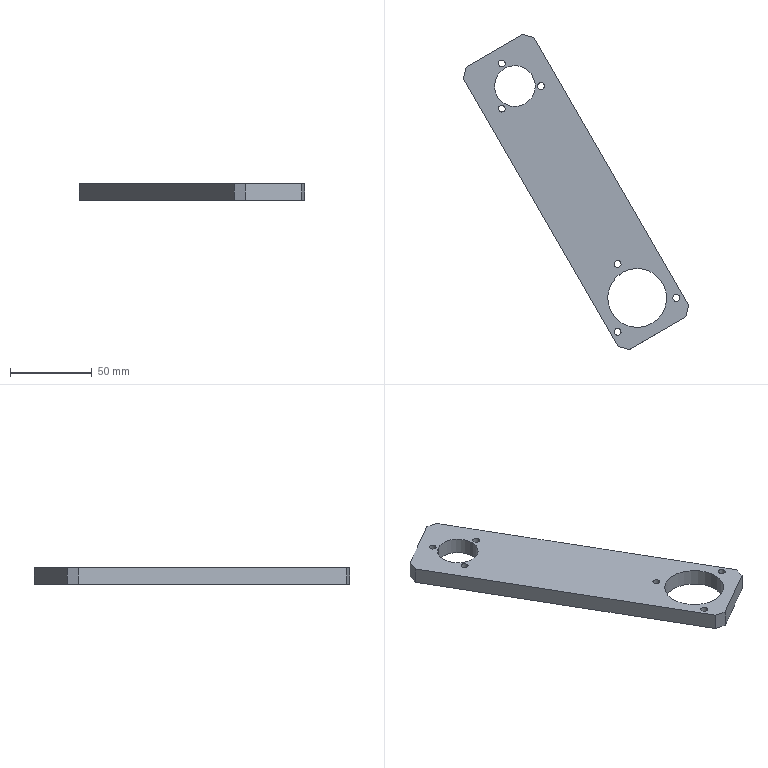Component | SolidWorks | JYTBJ-HeaderPlateSupportFrameA-1 | 1 solid | 26 faces | box 138.3 x 193.21 x 10 mm | volume 83525 mm3 | cylinder 16 | plane 10 | commonest cylinder face diameters 4.2 x12 36.1 x2 25 x2
build123d program:
from build123d import *

# Parameters (mm, degrees)
SKETCH1_W           = 200
SKETCH1_H           = 50
SKETCH1_R           = 12.5
SKETCH1_R_2         = 18.05
BOSS_EXTRUDE1_DEPTH = 10
M5_TAPPED_HOLE1_D   = 4.2
CIRPATTERN1_COUNT   = 3
M5_TAPPED_HOLE2_D   = 4.2
CIRPATTERN2_COUNT   = 3
CHAMFER1_SIZE       = 5


with BuildPart() as part:
    # Sketch1 → Boss-Extrude1 (new body)
    with BuildSketch(Plane.XY):
        with Locations((75, 0)):
            Rectangle(SKETCH1_W, SKETCH1_H)
        Circle(SKETCH1_R, mode=Mode.SUBTRACT)
        with Locations((150, 0)):
            Circle(SKETCH1_R_2, mode=Mode.SUBTRACT)
    extrude(amount=BOSS_EXTRUDE1_DEPTH)

    # M5 Tapped Hole1 (through all)
    with Locations(Plane.XY.offset(10)):
        with Locations((126, 0)):
            m5_tapped_hole1 = Hole(M5_TAPPED_HOLE1_D / 2)

    # CirPattern1: M5 Tapped Hole1 ×3 about axis
    cirpattern1_axis = Axis((150, 0, 0), (0, 0, 1))
    for i in range(1, CIRPATTERN1_COUNT):
        add(m5_tapped_hole1.rotate(cirpattern1_axis, i * 360 / CIRPATTERN1_COUNT), mode=Mode.SUBTRACT)

    # M5 Tapped Hole2 (through all)
    with Locations(Plane.XY.offset(10)):
        with Locations((-16, 0)):
            m5_tapped_hole2 = Hole(M5_TAPPED_HOLE2_D / 2)

    # CirPattern2: M5 Tapped Hole2 ×3 about axis
    cirpattern2_axis = Axis((0, 0, 0), (0, 0, 1))
    for i in range(1, CIRPATTERN2_COUNT):
        add(m5_tapped_hole2.rotate(cirpattern2_axis, i * 360 / CIRPATTERN2_COUNT), mode=Mode.SUBTRACT)

    # Chamfer1
    chamfer1_edges = [part.edges().sort_by_distance(p)[0] for p in [
        (175, -25, 5),
        (-25, -25, 5),
        (-25, 25, 5),
        (175, 25, 5),
    ]]
    chamfer(chamfer1_edges, length=CHAMFER1_SIZE)


solid = part.part

# Placed as in the assembly
solid = solid.moved(Location((-71.627, 226.781, -28), (0, 0, -60)))
STEP:
#1=CARTESIAN_POINT('',(-3.176,8.454,-1.102));
#2=VERTEX_POINT('',#1);
#3=CARTESIAN_POINT('',(-3.094,8.311,-1.102));
#4=VERTEX_POINT('',#3);
#5=CARTESIAN_POINT('',(-3.135,8.383,-1.102));
#6=DIRECTION('',(0.,0.,1.));
#7=DIRECTION('',(0.5,-0.866,0.));
#8=AXIS2_PLACEMENT_3D('',#5,#6,#7);
#9=CIRCLE('',#8,0.08268);
#10=EDGE_CURVE('',#2,#4,#9,.T.);
#11=ORIENTED_EDGE('',*,*,#10,.F.);
#12=CARTESIAN_POINT('',(-3.176,8.454,-0.7087));
#13=VERTEX_POINT('',#12);
#14=CARTESIAN_POINT('',(-3.176,8.454,-0.7087));
#15=DIRECTION('',(0.,0.,1.));
#16=VECTOR('',#15,39.37);
#17=LINE('',#14,#16);
#18=EDGE_CURVE('',#2,#13,#17,.T.);
#19=ORIENTED_EDGE('',*,*,#18,.T.);
#20=CARTESIAN_POINT('',(-3.094,8.311,-0.7087));
#21=VERTEX_POINT('',#20);
#22=CARTESIAN_POINT('',(-3.135,8.383,-0.7087));
#23=DIRECTION('',(0.,0.,1.));
#24=DIRECTION('',(0.5,-0.866,0.));
#25=AXIS2_PLACEMENT_3D('',#22,#23,#24);
#26=CIRCLE('',#25,0.08268);
#27=EDGE_CURVE('',#13,#21,#26,.T.);
#28=ORIENTED_EDGE('',*,*,#27,.T.);
#29=CARTESIAN_POINT('',(-3.094,8.311,-0.7087));
#30=DIRECTION('',(0.,0.,1.));
#31=VECTOR('',#30,39.37);
#32=LINE('',#29,#31);
#33=EDGE_CURVE('',#4,#21,#32,.T.);
#34=ORIENTED_EDGE('',*,*,#33,.F.);
#35=EDGE_LOOP('',(#11,#19,#28,#34));
#36=FACE_OUTER_BOUND('',#35,.T.);
#37=CARTESIAN_POINT('',(-3.135,8.383,-0.7087));
#38=DIRECTION('',(0.,0.,1.));
#39=DIRECTION('',(0.5,-0.866,0.));
#40=AXIS2_PLACEMENT_3D('',#37,#38,#39);
#41=CYLINDRICAL_SURFACE('',#40,0.08268);
#42=ADVANCED_FACE('',(#36),#41,.F.);
#43=CARTESIAN_POINT('',(-2.231,9.,-1.102));
#44=VERTEX_POINT('',#43);
#45=CARTESIAN_POINT('',(-2.149,8.857,-1.102));
#46=VERTEX_POINT('',#45);
#47=CARTESIAN_POINT('',(-2.19,8.928,-1.102));
#48=DIRECTION('',(0.,0.,1.));
#49=DIRECTION('',(0.5,-0.866,0.));
#50=AXIS2_PLACEMENT_3D('',#47,#48,#49);
#51=CIRCLE('',#50,0.08268);
#52=EDGE_CURVE('',#44,#46,#51,.T.);
#53=ORIENTED_EDGE('',*,*,#52,.F.);
#54=CARTESIAN_POINT('',(-2.231,9.,-0.7087));
#55=VERTEX_POINT('',#54);
#56=CARTESIAN_POINT('',(-2.231,9.,-0.7087));
#57=DIRECTION('',(0.,0.,1.));
#58=VECTOR('',#57,39.37);
#59=LINE('',#56,#58);
#60=EDGE_CURVE('',#44,#55,#59,.T.);
#61=ORIENTED_EDGE('',*,*,#60,.T.);
#62=CARTESIAN_POINT('',(-2.149,8.857,-0.7087));
#63=VERTEX_POINT('',#62);
#64=CARTESIAN_POINT('',(-2.19,8.928,-0.7087));
#65=DIRECTION('',(0.,0.,1.));
#66=DIRECTION('',(0.5,-0.866,0.));
#67=AXIS2_PLACEMENT_3D('',#64,#65,#66);
#68=CIRCLE('',#67,0.08268);
#69=EDGE_CURVE('',#55,#63,#68,.T.);
#70=ORIENTED_EDGE('',*,*,#69,.T.);
#71=CARTESIAN_POINT('',(-2.149,8.857,-0.7087));
#72=DIRECTION('',(0.,0.,1.));
#73=VECTOR('',#72,39.37);
#74=LINE('',#71,#73);
#75=EDGE_CURVE('',#46,#63,#74,.T.);
#76=ORIENTED_EDGE('',*,*,#75,.F.);
#77=EDGE_LOOP('',(#53,#61,#70,#76));
#78=FACE_OUTER_BOUND('',#77,.T.);
#79=CARTESIAN_POINT('',(-2.19,8.928,-0.7087));
#80=DIRECTION('',(0.,0.,1.));
#81=DIRECTION('',(0.5,-0.866,0.));
#82=AXIS2_PLACEMENT_3D('',#79,#80,#81);
#83=CYLINDRICAL_SURFACE('',#82,0.08268);
#84=ADVANCED_FACE('',(#78),#83,.F.);
#85=CARTESIAN_POINT('',(-3.176,9.546,-1.102));
#86=VERTEX_POINT('',#85);
#87=CARTESIAN_POINT('',(-3.094,9.402,-1.102));
#88=VERTEX_POINT('',#87);
#89=CARTESIAN_POINT('',(-3.135,9.474,-1.102));
#90=DIRECTION('',(0.,0.,1.));
#91=DIRECTION('',(0.5,-0.866,0.));
#92=AXIS2_PLACEMENT_3D('',#89,#90,#91);
#93=CIRCLE('',#92,0.08268);
#94=EDGE_CURVE('',#86,#88,#93,.T.);
#95=ORIENTED_EDGE('',*,*,#94,.F.);
#96=CARTESIAN_POINT('',(-3.176,9.546,-0.7087));
#97=VERTEX_POINT('',#96);
#98=CARTESIAN_POINT('',(-3.176,9.546,-0.7087));
#99=DIRECTION('',(0.,0.,1.));
#100=VECTOR('',#99,39.37);
#101=LINE('',#98,#100);
#102=EDGE_CURVE('',#86,#97,#101,.T.);
#103=ORIENTED_EDGE('',*,*,#102,.T.);
#104=CARTESIAN_POINT('',(-3.094,9.402,-0.7087));
#105=VERTEX_POINT('',#104);
#106=CARTESIAN_POINT('',(-3.135,9.474,-0.7087));
#107=DIRECTION('',(0.,0.,1.));
#108=DIRECTION('',(0.5,-0.866,0.));
#109=AXIS2_PLACEMENT_3D('',#106,#107,#108);
#110=CIRCLE('',#109,0.08268);
#111=EDGE_CURVE('',#97,#105,#110,.T.);
#112=ORIENTED_EDGE('',*,*,#111,.T.);
#113=CARTESIAN_POINT('',(-3.094,9.402,-0.7087));
#114=DIRECTION('',(0.,0.,1.));
#115=VECTOR('',#114,39.37);
#116=LINE('',#113,#115);
#117=EDGE_CURVE('',#88,#105,#116,.T.);
#118=ORIENTED_EDGE('',*,*,#117,.F.);
#119=EDGE_LOOP('',(#95,#103,#112,#118));
#120=FACE_OUTER_BOUND('',#119,.T.);
#121=CARTESIAN_POINT('',(-3.135,9.474,-0.7087));
#122=DIRECTION('',(0.,0.,1.));
#123=DIRECTION('',(0.5,-0.866,0.));
#124=AXIS2_PLACEMENT_3D('',#121,#122,#123);
#125=CYLINDRICAL_SURFACE('',#124,0.08268);
#126=ADVANCED_FACE('',(#120),#125,.F.);
#127=CARTESIAN_POINT('',(1.036,3.886,-1.102));
#128=VERTEX_POINT('',#127);
#129=CARTESIAN_POINT('',(1.119,3.742,-1.102));
#130=VERTEX_POINT('',#129);
#131=CARTESIAN_POINT('',(1.078,3.814,-1.102));
#132=DIRECTION('',(0.,0.,1.));
#133=DIRECTION('',(0.5,-0.866,0.));
#134=AXIS2_PLACEMENT_3D('',#131,#132,#133);
#135=CIRCLE('',#134,0.08268);
#136=EDGE_CURVE('',#128,#130,#135,.T.);
#137=ORIENTED_EDGE('',*,*,#136,.F.);
#138=CARTESIAN_POINT('',(1.036,3.886,-0.7087));
#139=VERTEX_POINT('',#138);
#140=CARTESIAN_POINT('',(1.036,3.886,-0.7087));
#141=DIRECTION('',(0.,0.,1.));
#142=VECTOR('',#141,39.37);
#143=LINE('',#140,#142);
#144=EDGE_CURVE('',#128,#139,#143,.T.);
#145=ORIENTED_EDGE('',*,*,#144,.T.);
#146=CARTESIAN_POINT('',(1.119,3.742,-0.7087));
#147=VERTEX_POINT('',#146);
#148=CARTESIAN_POINT('',(1.078,3.814,-0.7087));
#149=DIRECTION('',(0.,0.,1.));
#150=DIRECTION('',(0.5,-0.866,0.));
#151=AXIS2_PLACEMENT_3D('',#148,#149,#150);
#152=CIRCLE('',#151,0.08268);
#153=EDGE_CURVE('',#139,#147,#152,.T.);
#154=ORIENTED_EDGE('',*,*,#153,.T.);
#155=CARTESIAN_POINT('',(1.119,3.742,-0.7087));
#156=DIRECTION('',(0.,0.,1.));
#157=VECTOR('',#156,39.37);
#158=LINE('',#155,#157);
#159=EDGE_CURVE('',#130,#147,#158,.T.);
#160=ORIENTED_EDGE('',*,*,#159,.F.);
#161=EDGE_LOOP('',(#137,#145,#154,#160));
#162=FACE_OUTER_BOUND('',#161,.T.);
#163=CARTESIAN_POINT('',(1.078,3.814,-0.7087));
#164=DIRECTION('',(0.,0.,1.));
#165=DIRECTION('',(0.5,-0.866,0.));
#166=AXIS2_PLACEMENT_3D('',#163,#164,#165);
#167=CYLINDRICAL_SURFACE('',#166,0.08268);
#168=ADVANCED_FACE('',(#162),#167,.F.);
#169=CARTESIAN_POINT('',(-0.381,3.067,-1.102));
#170=VERTEX_POINT('',#169);
#171=CARTESIAN_POINT('',(-0.2983,2.924,-1.102));
#172=VERTEX_POINT('',#171);
#173=CARTESIAN_POINT('',(-0.3396,2.996,-1.102));
#174=DIRECTION('',(0.,0.,1.));
#175=DIRECTION('',(0.5,-0.866,0.));
#176=AXIS2_PLACEMENT_3D('',#173,#174,#175);
#177=CIRCLE('',#176,0.08268);
#178=EDGE_CURVE('',#170,#172,#177,.T.);
#179=ORIENTED_EDGE('',*,*,#178,.F.);
#180=CARTESIAN_POINT('',(-0.381,3.067,-0.7087));
#181=VERTEX_POINT('',#180);
#182=CARTESIAN_POINT('',(-0.381,3.067,-0.7087));
#183=DIRECTION('',(0.,0.,1.));
#184=VECTOR('',#183,39.37);
#185=LINE('',#182,#184);
#186=EDGE_CURVE('',#170,#181,#185,.T.);
#187=ORIENTED_EDGE('',*,*,#186,.T.);
#188=CARTESIAN_POINT('',(-0.2983,2.924,-0.7087));
#189=VERTEX_POINT('',#188);
#190=CARTESIAN_POINT('',(-0.3396,2.996,-0.7087));
#191=DIRECTION('',(0.,0.,1.));
#192=DIRECTION('',(0.5,-0.866,0.));
#193=AXIS2_PLACEMENT_3D('',#190,#191,#192);
#194=CIRCLE('',#193,0.08268);
#195=EDGE_CURVE('',#181,#189,#194,.T.);
#196=ORIENTED_EDGE('',*,*,#195,.T.);
#197=CARTESIAN_POINT('',(-0.2983,2.924,-0.7087));
#198=DIRECTION('',(0.,0.,1.));
#199=VECTOR('',#198,39.37);
#200=LINE('',#197,#199);
#201=EDGE_CURVE('',#172,#189,#200,.T.);
#202=ORIENTED_EDGE('',*,*,#201,.F.);
#203=EDGE_LOOP('',(#179,#187,#196,#202));
#204=FACE_OUTER_BOUND('',#203,.T.);
#205=CARTESIAN_POINT('',(-0.3396,2.996,-0.7087));
#206=DIRECTION('',(0.,0.,1.));
#207=DIRECTION('',(0.5,-0.866,0.));
#208=AXIS2_PLACEMENT_3D('',#205,#206,#207);
#209=CYLINDRICAL_SURFACE('',#208,0.08268);
#210=ADVANCED_FACE('',(#204),#209,.F.);
#211=CARTESIAN_POINT('',(-0.381,4.704,-1.102));
#212=VERTEX_POINT('',#211);
#213=CARTESIAN_POINT('',(-0.2983,4.561,-1.102));
#214=VERTEX_POINT('',#213);
#215=CARTESIAN_POINT('',(-0.3396,4.632,-1.102));
#216=DIRECTION('',(0.,0.,1.));
#217=DIRECTION('',(0.5,-0.866,0.));
#218=AXIS2_PLACEMENT_3D('',#215,#216,#217);
#219=CIRCLE('',#218,0.08268);
#220=EDGE_CURVE('',#212,#214,#219,.T.);
#221=ORIENTED_EDGE('',*,*,#220,.F.);
#222=CARTESIAN_POINT('',(-0.381,4.704,-0.7087));
#223=VERTEX_POINT('',#222);
#224=CARTESIAN_POINT('',(-0.381,4.704,-0.7087));
#225=DIRECTION('',(0.,0.,1.));
#226=VECTOR('',#225,39.37);
#227=LINE('',#224,#226);
#228=EDGE_CURVE('',#212,#223,#227,.T.);
#229=ORIENTED_EDGE('',*,*,#228,.T.);
#230=CARTESIAN_POINT('',(-0.2983,4.561,-0.7087));
#231=VERTEX_POINT('',#230);
#232=CARTESIAN_POINT('',(-0.3396,4.632,-0.7087));
#233=DIRECTION('',(0.,0.,1.));
#234=DIRECTION('',(0.5,-0.866,0.));
#235=AXIS2_PLACEMENT_3D('',#232,#233,#234);
#236=CIRCLE('',#235,0.08268);
#237=EDGE_CURVE('',#223,#231,#236,.T.);
#238=ORIENTED_EDGE('',*,*,#237,.T.);
#239=CARTESIAN_POINT('',(-0.2983,4.561,-0.7087));
#240=DIRECTION('',(0.,0.,1.));
#241=VECTOR('',#240,39.37);
#242=LINE('',#239,#241);
#243=EDGE_CURVE('',#214,#231,#242,.T.);
#244=ORIENTED_EDGE('',*,*,#243,.F.);
#245=EDGE_LOOP('',(#221,#229,#238,#244));
#246=FACE_OUTER_BOUND('',#245,.T.);
#247=CARTESIAN_POINT('',(-0.3396,4.632,-0.7087));
#248=DIRECTION('',(0.,0.,1.));
#249=DIRECTION('',(0.5,-0.866,0.));
#250=AXIS2_PLACEMENT_3D('',#247,#248,#249);
#251=CYLINDRICAL_SURFACE('',#250,0.08268);
#252=ADVANCED_FACE('',(#246),#251,.F.);
#253=CARTESIAN_POINT('',(-0.2225,4.43,-0.7087));
#254=VERTEX_POINT('',#253);
#255=CARTESIAN_POINT('',(0.4881,3.199,-0.7087));
#256=VERTEX_POINT('',#255);
#257=CARTESIAN_POINT('',(0.1328,3.814,-0.7087));
#258=DIRECTION('',(0.,0.,1.));
#259=DIRECTION('',(0.5,-0.866,0.));
#260=AXIS2_PLACEMENT_3D('',#257,#258,#259);
#261=CIRCLE('',#260,0.7106);
#262=EDGE_CURVE('',#254,#256,#261,.T.);
#263=ORIENTED_EDGE('',*,*,#262,.T.);
#264=CARTESIAN_POINT('',(0.4881,3.199,-1.102));
#265=VERTEX_POINT('',#264);
#266=CARTESIAN_POINT('',(0.4881,3.199,-0.7087));
#267=DIRECTION('',(0.,0.,-1.));
#268=VECTOR('',#267,39.37);
#269=LINE('',#266,#268);
#270=EDGE_CURVE('',#256,#265,#269,.T.);
#271=ORIENTED_EDGE('',*,*,#270,.T.);
#272=CARTESIAN_POINT('',(-0.2225,4.43,-1.102));
#273=VERTEX_POINT('',#272);
#274=CARTESIAN_POINT('',(0.1328,3.814,-1.102));
#275=DIRECTION('',(0.,0.,1.));
#276=DIRECTION('',(0.5,-0.866,0.));
#277=AXIS2_PLACEMENT_3D('',#274,#275,#276);
#278=CIRCLE('',#277,0.7106);
#279=EDGE_CURVE('',#273,#265,#278,.T.);
#280=ORIENTED_EDGE('',*,*,#279,.F.);
#281=CARTESIAN_POINT('',(-0.2225,4.43,-0.7087));
#282=DIRECTION('',(0.,0.,-1.));
#283=VECTOR('',#282,39.37);
#284=LINE('',#281,#283);
#285=EDGE_CURVE('',#254,#273,#284,.T.);
#286=ORIENTED_EDGE('',*,*,#285,.F.);
#287=EDGE_LOOP('',(#263,#271,#280,#286));
#288=FACE_OUTER_BOUND('',#287,.T.);
#289=CARTESIAN_POINT('',(0.1328,3.814,-0.7087));
#290=DIRECTION('',(0.,0.,-1.));
#291=DIRECTION('',(-0.5,0.866,0.));
#292=AXIS2_PLACEMENT_3D('',#289,#290,#291);
#293=CYLINDRICAL_SURFACE('',#292,0.7106);
#294=ADVANCED_FACE('',(#288),#293,.F.);
#295=CARTESIAN_POINT('',(-3.066,9.355,-0.7087));
#296=VERTEX_POINT('',#295);
#297=CARTESIAN_POINT('',(-2.574,8.502,-0.7087));
#298=VERTEX_POINT('',#297);
#299=CARTESIAN_POINT('',(-2.82,8.928,-0.7087));
#300=DIRECTION('',(0.,0.,1.));
#301=DIRECTION('',(0.5,-0.866,0.));
#302=AXIS2_PLACEMENT_3D('',#299,#300,#301);
#303=CIRCLE('',#302,0.4921);
#304=EDGE_CURVE('',#296,#298,#303,.T.);
#305=ORIENTED_EDGE('',*,*,#304,.T.);
#306=CARTESIAN_POINT('',(-2.574,8.502,-1.102));
#307=VERTEX_POINT('',#306);
#308=CARTESIAN_POINT('',(-2.574,8.502,-0.7087));
#309=DIRECTION('',(0.,0.,-1.));
#310=VECTOR('',#309,39.37);
#311=LINE('',#308,#310);
#312=EDGE_CURVE('',#298,#307,#311,.T.);
#313=ORIENTED_EDGE('',*,*,#312,.T.);
#314=CARTESIAN_POINT('',(-3.066,9.355,-1.102));
#315=VERTEX_POINT('',#314);
#316=CARTESIAN_POINT('',(-2.82,8.928,-1.102));
#317=DIRECTION('',(0.,0.,1.));
#318=DIRECTION('',(0.5,-0.866,0.));
#319=AXIS2_PLACEMENT_3D('',#316,#317,#318);
#320=CIRCLE('',#319,0.4921);
#321=EDGE_CURVE('',#315,#307,#320,.T.);
#322=ORIENTED_EDGE('',*,*,#321,.F.);
#323=CARTESIAN_POINT('',(-3.066,9.355,-0.7087));
#324=DIRECTION('',(0.,0.,-1.));
#325=VECTOR('',#324,39.37);
#326=LINE('',#323,#325);
#327=EDGE_CURVE('',#296,#315,#326,.T.);
#328=ORIENTED_EDGE('',*,*,#327,.F.);
#329=EDGE_LOOP('',(#305,#313,#322,#328));
#330=FACE_OUTER_BOUND('',#329,.T.);
#331=CARTESIAN_POINT('',(-2.82,8.928,-0.7087));
#332=DIRECTION('',(0.,0.,-1.));
#333=DIRECTION('',(-0.5,0.866,0.));
#334=AXIS2_PLACEMENT_3D('',#331,#332,#333);
#335=CYLINDRICAL_SURFACE('',#334,0.4921);
#336=ADVANCED_FACE('',(#330),#335,.F.);
#337=CARTESIAN_POINT('',(-3.135,8.383,-0.7087));
#338=DIRECTION('',(0.,0.,1.));
#339=DIRECTION('',(0.5,-0.866,0.));
#340=AXIS2_PLACEMENT_3D('',#337,#338,#339);
#341=CIRCLE('',#340,0.08268);
#342=EDGE_CURVE('',#21,#13,#341,.T.);
#343=ORIENTED_EDGE('',*,*,#342,.F.);
#344=ORIENTED_EDGE('',*,*,#27,.F.);
#345=EDGE_LOOP('',(#343,#344));
#346=FACE_BOUND('',#345,.T.);
#347=CARTESIAN_POINT('',(-2.19,8.928,-0.7087));
#348=DIRECTION('',(0.,0.,1.));
#349=DIRECTION('',(0.5,-0.866,0.));
#350=AXIS2_PLACEMENT_3D('',#347,#348,#349);
#351=CIRCLE('',#350,0.08268);
#352=EDGE_CURVE('',#63,#55,#351,.T.);
#353=ORIENTED_EDGE('',*,*,#352,.F.);
#354=ORIENTED_EDGE('',*,*,#69,.F.);
#355=EDGE_LOOP('',(#353,#354));
#356=FACE_BOUND('',#355,.T.);
#357=CARTESIAN_POINT('',(-3.135,9.474,-0.7087));
#358=DIRECTION('',(0.,0.,1.));
#359=DIRECTION('',(0.5,-0.866,0.));
#360=AXIS2_PLACEMENT_3D('',#357,#358,#359);
#361=CIRCLE('',#360,0.08268);
#362=EDGE_CURVE('',#105,#97,#361,.T.);
#363=ORIENTED_EDGE('',*,*,#362,.F.);
#364=ORIENTED_EDGE('',*,*,#111,.F.);
#365=EDGE_LOOP('',(#363,#364));
#366=FACE_BOUND('',#365,.T.);
#367=CARTESIAN_POINT('',(1.078,3.814,-0.7087));
#368=DIRECTION('',(0.,0.,1.));
#369=DIRECTION('',(0.5,-0.866,0.));
#370=AXIS2_PLACEMENT_3D('',#367,#368,#369);
#371=CIRCLE('',#370,0.08268);
#372=EDGE_CURVE('',#147,#139,#371,.T.);
#373=ORIENTED_EDGE('',*,*,#372,.F.);
#374=ORIENTED_EDGE('',*,*,#153,.F.);
#375=EDGE_LOOP('',(#373,#374));
#376=FACE_BOUND('',#375,.T.);
#377=CARTESIAN_POINT('',(-0.3396,2.996,-0.7087));
#378=DIRECTION('',(0.,0.,1.));
#379=DIRECTION('',(0.5,-0.866,0.));
#380=AXIS2_PLACEMENT_3D('',#377,#378,#379);
#381=CIRCLE('',#380,0.08268);
#382=EDGE_CURVE('',#189,#181,#381,.T.);
#383=ORIENTED_EDGE('',*,*,#382,.F.);
#384=ORIENTED_EDGE('',*,*,#195,.F.);
#385=EDGE_LOOP('',(#383,#384));
#386=FACE_BOUND('',#385,.T.);
#387=CARTESIAN_POINT('',(-0.3396,4.632,-0.7087));
#388=DIRECTION('',(0.,0.,1.));
#389=DIRECTION('',(0.5,-0.866,0.));
#390=AXIS2_PLACEMENT_3D('',#387,#388,#389);
#391=CIRCLE('',#390,0.08268);
#392=EDGE_CURVE('',#231,#223,#391,.T.);
#393=ORIENTED_EDGE('',*,*,#392,.F.);
#394=ORIENTED_EDGE('',*,*,#237,.F.);
#395=EDGE_LOOP('',(#393,#394));
#396=FACE_BOUND('',#395,.T.);
#397=ORIENTED_EDGE('',*,*,#304,.F.);
#398=CARTESIAN_POINT('',(-2.82,8.928,-0.7087));
#399=DIRECTION('',(0.,0.,1.));
#400=DIRECTION('',(0.5,-0.866,0.));
#401=AXIS2_PLACEMENT_3D('',#398,#399,#400);
#402=CIRCLE('',#401,0.4921);
#403=EDGE_CURVE('',#298,#296,#402,.T.);
#404=ORIENTED_EDGE('',*,*,#403,.F.);
#405=EDGE_LOOP('',(#397,#404));
#406=FACE_BOUND('',#405,.T.);
#407=CARTESIAN_POINT('',(-4.066,9.118,-0.7087));
#408=VERTEX_POINT('',#407);
#409=CARTESIAN_POINT('',(-0.3259,2.64,-0.7087));
#410=VERTEX_POINT('',#409);
#411=CARTESIAN_POINT('',(-4.164,9.289,-0.7087));
#412=DIRECTION('',(0.5,-0.866,0.));
#413=VECTOR('',#412,39.37);
#414=LINE('',#411,#413);
#415=EDGE_CURVE('',#408,#410,#414,.T.);
#416=ORIENTED_EDGE('',*,*,#415,.T.);
#417=CARTESIAN_POINT('',(-0.05697,2.568,-0.7087));
#418=VERTEX_POINT('',#417);
#419=CARTESIAN_POINT('',(-0.1914,2.604,-0.7087));
#420=DIRECTION('',(0.9659,-0.2588,0.));
#421=VECTOR('',#420,39.37);
#422=LINE('',#419,#421);
#423=EDGE_CURVE('',#410,#418,#422,.T.);
#424=ORIENTED_EDGE('',*,*,#423,.T.);
#425=CARTESIAN_POINT('',(1.307,3.355,-0.7087));
#426=VERTEX_POINT('',#425);
#427=CARTESIAN_POINT('',(1.477,3.454,-0.7087));
#428=DIRECTION('',(0.866,0.5,0.));
#429=VECTOR('',#428,39.37);
#430=LINE('',#427,#429);
#431=EDGE_CURVE('',#418,#426,#430,.T.);
#432=ORIENTED_EDGE('',*,*,#431,.T.);
#433=CARTESIAN_POINT('',(1.379,3.624,-0.7087));
#434=VERTEX_POINT('',#433);
#435=CARTESIAN_POINT('',(0.9826,2.145,-0.7087));
#436=DIRECTION('',(0.2588,0.9659,0.));
#437=VECTOR('',#436,39.37);
#438=LINE('',#435,#437);
#439=EDGE_CURVE('',#426,#434,#438,.T.);
#440=ORIENTED_EDGE('',*,*,#439,.T.);
#441=CARTESIAN_POINT('',(-2.361,10.102,-0.7087));
#442=VERTEX_POINT('',#441);
#443=CARTESIAN_POINT('',(-2.46,10.273,-0.7087));
#444=DIRECTION('',(-0.5,0.866,0.));
#445=VECTOR('',#444,39.37);
#446=LINE('',#443,#445);
#447=EDGE_CURVE('',#434,#442,#446,.T.);
#448=ORIENTED_EDGE('',*,*,#447,.T.);
#449=CARTESIAN_POINT('',(-2.63,10.174,-0.7087));
#450=VERTEX_POINT('',#449);
#451=CARTESIAN_POINT('',(1.538,9.058,-0.7087));
#452=DIRECTION('',(-0.9659,0.2588,0.));
#453=VECTOR('',#452,39.37);
#454=LINE('',#451,#453);
#455=EDGE_CURVE('',#442,#450,#454,.T.);
#456=ORIENTED_EDGE('',*,*,#455,.T.);
#457=CARTESIAN_POINT('',(-3.994,9.387,-0.7087));
#458=VERTEX_POINT('',#457);
#459=CARTESIAN_POINT('',(-4.164,9.289,-0.7087));
#460=DIRECTION('',(-0.866,-0.5,0.));
#461=VECTOR('',#460,39.37);
#462=LINE('',#459,#461);
#463=EDGE_CURVE('',#450,#458,#462,.T.);
#464=ORIENTED_EDGE('',*,*,#463,.T.);
#465=CARTESIAN_POINT('',(-5.471,3.875,-0.7087));
#466=DIRECTION('',(-0.2588,-0.9659,0.));
#467=VECTOR('',#466,39.37);
#468=LINE('',#465,#467);
#469=EDGE_CURVE('',#458,#408,#468,.T.);
#470=ORIENTED_EDGE('',*,*,#469,.T.);
#471=EDGE_LOOP('',(#416,#424,#432,#440,#448,#456,#464,#470));
#472=FACE_OUTER_BOUND('',#471,.T.);
#473=ORIENTED_EDGE('',*,*,#262,.F.);
#474=CARTESIAN_POINT('',(0.1328,3.814,-0.7087));
#475=DIRECTION('',(0.,0.,1.));
#476=DIRECTION('',(0.5,-0.866,0.));
#477=AXIS2_PLACEMENT_3D('',#474,#475,#476);
#478=CIRCLE('',#477,0.7106);
#479=EDGE_CURVE('',#256,#254,#478,.T.);
#480=ORIENTED_EDGE('',*,*,#479,.F.);
#481=EDGE_LOOP('',(#473,#480));
#482=FACE_BOUND('',#481,.T.);
#483=CARTESIAN_POINT('',(-0.2274,2.47,-0.7087));
#484=DIRECTION('',(0.,0.,1.));
#485=DIRECTION('',(0.5,-0.866,0.));
#486=AXIS2_PLACEMENT_3D('',#483,#484,#485);
#487=PLANE('',#486);
#488=ADVANCED_FACE('',(#346,#356,#366,#376,#386,#396,#406,#472,#482),#487,.T.);
#489=CARTESIAN_POINT('',(-3.135,8.383,-1.102));
#490=DIRECTION('',(0.,0.,1.));
#491=DIRECTION('',(0.5,-0.866,0.));
#492=AXIS2_PLACEMENT_3D('',#489,#490,#491);
#493=CIRCLE('',#492,0.08268);
#494=EDGE_CURVE('',#4,#2,#493,.T.);
#495=ORIENTED_EDGE('',*,*,#494,.T.);
#496=ORIENTED_EDGE('',*,*,#10,.T.);
#497=EDGE_LOOP('',(#495,#496));
#498=FACE_BOUND('',#497,.T.);
#499=CARTESIAN_POINT('',(-2.19,8.928,-1.102));
#500=DIRECTION('',(0.,0.,1.));
#501=DIRECTION('',(0.5,-0.866,0.));
#502=AXIS2_PLACEMENT_3D('',#499,#500,#501);
#503=CIRCLE('',#502,0.08268);
#504=EDGE_CURVE('',#46,#44,#503,.T.);
#505=ORIENTED_EDGE('',*,*,#504,.T.);
#506=ORIENTED_EDGE('',*,*,#52,.T.);
#507=EDGE_LOOP('',(#505,#506));
#508=FACE_BOUND('',#507,.T.);
#509=CARTESIAN_POINT('',(-3.135,9.474,-1.102));
#510=DIRECTION('',(0.,0.,1.));
#511=DIRECTION('',(0.5,-0.866,0.));
#512=AXIS2_PLACEMENT_3D('',#509,#510,#511);
#513=CIRCLE('',#512,0.08268);
#514=EDGE_CURVE('',#88,#86,#513,.T.);
#515=ORIENTED_EDGE('',*,*,#514,.T.);
#516=ORIENTED_EDGE('',*,*,#94,.T.);
#517=EDGE_LOOP('',(#515,#516));
#518=FACE_BOUND('',#517,.T.);
#519=CARTESIAN_POINT('',(1.078,3.814,-1.102));
#520=DIRECTION('',(0.,0.,1.));
#521=DIRECTION('',(0.5,-0.866,0.));
#522=AXIS2_PLACEMENT_3D('',#519,#520,#521);
#523=CIRCLE('',#522,0.08268);
#524=EDGE_CURVE('',#130,#128,#523,.T.);
#525=ORIENTED_EDGE('',*,*,#524,.T.);
#526=ORIENTED_EDGE('',*,*,#136,.T.);
#527=EDGE_LOOP('',(#525,#526));
#528=FACE_BOUND('',#527,.T.);
#529=CARTESIAN_POINT('',(-0.3396,2.996,-1.102));
#530=DIRECTION('',(0.,0.,1.));
#531=DIRECTION('',(0.5,-0.866,0.));
#532=AXIS2_PLACEMENT_3D('',#529,#530,#531);
#533=CIRCLE('',#532,0.08268);
#534=EDGE_CURVE('',#172,#170,#533,.T.);
#535=ORIENTED_EDGE('',*,*,#534,.T.);
#536=ORIENTED_EDGE('',*,*,#178,.T.);
#537=EDGE_LOOP('',(#535,#536));
#538=FACE_BOUND('',#537,.T.);
#539=CARTESIAN_POINT('',(-0.3396,4.632,-1.102));
#540=DIRECTION('',(0.,0.,1.));
#541=DIRECTION('',(0.5,-0.866,0.));
#542=AXIS2_PLACEMENT_3D('',#539,#540,#541);
#543=CIRCLE('',#542,0.08268);
#544=EDGE_CURVE('',#214,#212,#543,.T.);
#545=ORIENTED_EDGE('',*,*,#544,.T.);
#546=ORIENTED_EDGE('',*,*,#220,.T.);
#547=EDGE_LOOP('',(#545,#546));
#548=FACE_BOUND('',#547,.T.);
#549=ORIENTED_EDGE('',*,*,#321,.T.);
#550=CARTESIAN_POINT('',(-2.82,8.928,-1.102));
#551=DIRECTION('',(0.,0.,1.));
#552=DIRECTION('',(0.5,-0.866,0.));
#553=AXIS2_PLACEMENT_3D('',#550,#551,#552);
#554=CIRCLE('',#553,0.4921);
#555=EDGE_CURVE('',#307,#315,#554,.T.);
#556=ORIENTED_EDGE('',*,*,#555,.T.);
#557=EDGE_LOOP('',(#549,#556));
#558=FACE_BOUND('',#557,.T.);
#559=CARTESIAN_POINT('',(-0.05697,2.568,-1.102));
#560=VERTEX_POINT('',#559);
#561=CARTESIAN_POINT('',(1.307,3.355,-1.102));
#562=VERTEX_POINT('',#561);
#563=CARTESIAN_POINT('',(1.477,3.454,-1.102));
#564=DIRECTION('',(0.866,0.5,0.));
#565=VECTOR('',#564,39.37);
#566=LINE('',#563,#565);
#567=EDGE_CURVE('',#560,#562,#566,.T.);
#568=ORIENTED_EDGE('',*,*,#567,.F.);
#569=CARTESIAN_POINT('',(-0.3259,2.64,-1.102));
#570=VERTEX_POINT('',#569);
#571=CARTESIAN_POINT('',(-0.05697,2.568,-1.102));
#572=DIRECTION('',(-0.9659,0.2588,0.));
#573=VECTOR('',#572,39.37);
#574=LINE('',#571,#573);
#575=EDGE_CURVE('',#560,#570,#574,.T.);
#576=ORIENTED_EDGE('',*,*,#575,.T.);
#577=CARTESIAN_POINT('',(-4.066,9.118,-1.102));
#578=VERTEX_POINT('',#577);
#579=CARTESIAN_POINT('',(-4.164,9.289,-1.102));
#580=DIRECTION('',(0.5,-0.866,0.));
#581=VECTOR('',#580,39.37);
#582=LINE('',#579,#581);
#583=EDGE_CURVE('',#578,#570,#582,.T.);
#584=ORIENTED_EDGE('',*,*,#583,.F.);
#585=CARTESIAN_POINT('',(-3.994,9.387,-1.102));
#586=VERTEX_POINT('',#585);
#587=CARTESIAN_POINT('',(-4.066,9.118,-1.102));
#588=DIRECTION('',(0.2588,0.9659,0.));
#589=VECTOR('',#588,39.37);
#590=LINE('',#587,#589);
#591=EDGE_CURVE('',#578,#586,#590,.T.);
#592=ORIENTED_EDGE('',*,*,#591,.T.);
#593=CARTESIAN_POINT('',(-2.63,10.174,-1.102));
#594=VERTEX_POINT('',#593);
#595=CARTESIAN_POINT('',(-4.164,9.289,-1.102));
#596=DIRECTION('',(-0.866,-0.5,0.));
#597=VECTOR('',#596,39.37);
#598=LINE('',#595,#597);
#599=EDGE_CURVE('',#594,#586,#598,.T.);
#600=ORIENTED_EDGE('',*,*,#599,.F.);
#601=CARTESIAN_POINT('',(-2.361,10.102,-1.102));
#602=VERTEX_POINT('',#601);
#603=CARTESIAN_POINT('',(-2.63,10.174,-1.102));
#604=DIRECTION('',(0.9659,-0.2588,0.));
#605=VECTOR('',#604,39.37);
#606=LINE('',#603,#605);
#607=EDGE_CURVE('',#594,#602,#606,.T.);
#608=ORIENTED_EDGE('',*,*,#607,.T.);
#609=CARTESIAN_POINT('',(1.379,3.624,-1.102));
#610=VERTEX_POINT('',#609);
#611=CARTESIAN_POINT('',(-2.46,10.273,-1.102));
#612=DIRECTION('',(-0.5,0.866,0.));
#613=VECTOR('',#612,39.37);
#614=LINE('',#611,#613);
#615=EDGE_CURVE('',#610,#602,#614,.T.);
#616=ORIENTED_EDGE('',*,*,#615,.F.);
#617=CARTESIAN_POINT('',(1.379,3.624,-1.102));
#618=DIRECTION('',(-0.2588,-0.9659,0.));
#619=VECTOR('',#618,39.37);
#620=LINE('',#617,#619);
#621=EDGE_CURVE('',#610,#562,#620,.T.);
#622=ORIENTED_EDGE('',*,*,#621,.T.);
#623=EDGE_LOOP('',(#568,#576,#584,#592,#600,#608,#616,#622));
#624=FACE_OUTER_BOUND('',#623,.T.);
#625=ORIENTED_EDGE('',*,*,#279,.T.);
#626=CARTESIAN_POINT('',(0.1328,3.814,-1.102));
#627=DIRECTION('',(0.,0.,1.));
#628=DIRECTION('',(0.5,-0.866,0.));
#629=AXIS2_PLACEMENT_3D('',#626,#627,#628);
#630=CIRCLE('',#629,0.7106);
#631=EDGE_CURVE('',#265,#273,#630,.T.);
#632=ORIENTED_EDGE('',*,*,#631,.T.);
#633=EDGE_LOOP('',(#625,#632));
#634=FACE_BOUND('',#633,.T.);
#635=CARTESIAN_POINT('',(-0.2274,2.47,-1.102));
#636=DIRECTION('',(0.,0.,1.));
#637=DIRECTION('',(0.5,-0.866,0.));
#638=AXIS2_PLACEMENT_3D('',#635,#636,#637);
#639=PLANE('',#638);
#640=ADVANCED_FACE('',(#498,#508,#518,#528,#538,#548,#558,#624,#634),#639,.F.);
#641=ORIENTED_EDGE('',*,*,#431,.F.);
#642=CARTESIAN_POINT('',(-0.05697,2.568,-0.7087));
#643=DIRECTION('',(0.,0.,-1.));
#644=VECTOR('',#643,39.37);
#645=LINE('',#642,#644);
#646=EDGE_CURVE('',#418,#560,#645,.T.);
#647=ORIENTED_EDGE('',*,*,#646,.T.);
#648=ORIENTED_EDGE('',*,*,#567,.T.);
#649=CARTESIAN_POINT('',(1.307,3.355,-0.7087));
#650=DIRECTION('',(0.,0.,1.));
#651=VECTOR('',#650,39.37);
#652=LINE('',#649,#651);
#653=EDGE_CURVE('',#562,#426,#652,.T.);
#654=ORIENTED_EDGE('',*,*,#653,.T.);
#655=EDGE_LOOP('',(#641,#647,#648,#654));
#656=FACE_OUTER_BOUND('',#655,.T.);
#657=CARTESIAN_POINT('',(1.477,3.454,-0.7087));
#658=DIRECTION('',(-0.5,0.866,0.));
#659=DIRECTION('',(0.,0.,1.));
#660=AXIS2_PLACEMENT_3D('',#657,#658,#659);
#661=PLANE('',#660);
#662=ADVANCED_FACE('',(#656),#661,.F.);
#663=ORIENTED_EDGE('',*,*,#447,.F.);
#664=CARTESIAN_POINT('',(1.379,3.624,-0.7087));
#665=DIRECTION('',(0.,0.,-1.));
#666=VECTOR('',#665,39.37);
#667=LINE('',#664,#666);
#668=EDGE_CURVE('',#434,#610,#667,.T.);
#669=ORIENTED_EDGE('',*,*,#668,.T.);
#670=ORIENTED_EDGE('',*,*,#615,.T.);
#671=CARTESIAN_POINT('',(-2.361,10.102,-0.7087));
#672=DIRECTION('',(0.,0.,1.));
#673=VECTOR('',#672,39.37);
#674=LINE('',#671,#673);
#675=EDGE_CURVE('',#602,#442,#674,.T.);
#676=ORIENTED_EDGE('',*,*,#675,.T.);
#677=EDGE_LOOP('',(#663,#669,#670,#676));
#678=FACE_OUTER_BOUND('',#677,.T.);
#679=CARTESIAN_POINT('',(-2.46,10.273,-0.7087));
#680=DIRECTION('',(-0.866,-0.5,0.));
#681=DIRECTION('',(0.5,-0.866,0.));
#682=AXIS2_PLACEMENT_3D('',#679,#680,#681);
#683=PLANE('',#682);
#684=ADVANCED_FACE('',(#678),#683,.F.);
#685=ORIENTED_EDGE('',*,*,#599,.T.);
#686=CARTESIAN_POINT('',(-3.994,9.387,-0.7087));
#687=DIRECTION('',(0.,0.,1.));
#688=VECTOR('',#687,39.37);
#689=LINE('',#686,#688);
#690=EDGE_CURVE('',#586,#458,#689,.T.);
#691=ORIENTED_EDGE('',*,*,#690,.T.);
#692=ORIENTED_EDGE('',*,*,#463,.F.);
#693=CARTESIAN_POINT('',(-2.63,10.174,-0.7087));
#694=DIRECTION('',(0.,0.,-1.));
#695=VECTOR('',#694,39.37);
#696=LINE('',#693,#695);
#697=EDGE_CURVE('',#450,#594,#696,.T.);
#698=ORIENTED_EDGE('',*,*,#697,.T.);
#699=EDGE_LOOP('',(#685,#691,#692,#698));
#700=FACE_OUTER_BOUND('',#699,.T.);
#701=CARTESIAN_POINT('',(-4.164,9.289,-0.7087));
#702=DIRECTION('',(0.5,-0.866,0.));
#703=DIRECTION('',(0.866,0.5,0.));
#704=AXIS2_PLACEMENT_3D('',#701,#702,#703);
#705=PLANE('',#704);
#706=ADVANCED_FACE('',(#700),#705,.F.);
#707=ORIENTED_EDGE('',*,*,#583,.T.);
#708=CARTESIAN_POINT('',(-0.3259,2.64,-0.7087));
#709=DIRECTION('',(0.,0.,1.));
#710=VECTOR('',#709,39.37);
#711=LINE('',#708,#710);
#712=EDGE_CURVE('',#570,#410,#711,.T.);
#713=ORIENTED_EDGE('',*,*,#712,.T.);
#714=ORIENTED_EDGE('',*,*,#415,.F.);
#715=CARTESIAN_POINT('',(-4.066,9.118,-0.7087));
#716=DIRECTION('',(0.,0.,-1.));
#717=VECTOR('',#716,39.37);
#718=LINE('',#715,#717);
#719=EDGE_CURVE('',#408,#578,#718,.T.);
#720=ORIENTED_EDGE('',*,*,#719,.T.);
#721=EDGE_LOOP('',(#707,#713,#714,#720));
#722=FACE_OUTER_BOUND('',#721,.T.);
#723=CARTESIAN_POINT('',(-4.164,9.289,-0.7087));
#724=DIRECTION('',(0.866,0.5,0.));
#725=DIRECTION('',(-0.5,0.866,0.));
#726=AXIS2_PLACEMENT_3D('',#723,#724,#725);
#727=PLANE('',#726);
#728=ADVANCED_FACE('',(#722),#727,.F.);
#729=ORIENTED_EDGE('',*,*,#312,.F.);
#730=ORIENTED_EDGE('',*,*,#403,.T.);
#731=ORIENTED_EDGE('',*,*,#327,.T.);
#732=ORIENTED_EDGE('',*,*,#555,.F.);
#733=EDGE_LOOP('',(#729,#730,#731,#732));
#734=FACE_OUTER_BOUND('',#733,.T.);
#735=CARTESIAN_POINT('',(-2.82,8.928,-0.7087));
#736=DIRECTION('',(0.,0.,-1.));
#737=DIRECTION('',(-0.5,0.866,0.));
#738=AXIS2_PLACEMENT_3D('',#735,#736,#737);
#739=CYLINDRICAL_SURFACE('',#738,0.4921);
#740=ADVANCED_FACE('',(#734),#739,.F.);
#741=ORIENTED_EDGE('',*,*,#270,.F.);
#742=ORIENTED_EDGE('',*,*,#479,.T.);
#743=ORIENTED_EDGE('',*,*,#285,.T.);
#744=ORIENTED_EDGE('',*,*,#631,.F.);
#745=EDGE_LOOP('',(#741,#742,#743,#744));
#746=FACE_OUTER_BOUND('',#745,.T.);
#747=CARTESIAN_POINT('',(0.1328,3.814,-0.7087));
#748=DIRECTION('',(0.,0.,-1.));
#749=DIRECTION('',(-0.5,0.866,0.));
#750=AXIS2_PLACEMENT_3D('',#747,#748,#749);
#751=CYLINDRICAL_SURFACE('',#750,0.7106);
#752=ADVANCED_FACE('',(#746),#751,.F.);
#753=ORIENTED_EDGE('',*,*,#228,.F.);
#754=ORIENTED_EDGE('',*,*,#544,.F.);
#755=ORIENTED_EDGE('',*,*,#243,.T.);
#756=ORIENTED_EDGE('',*,*,#392,.T.);
#757=EDGE_LOOP('',(#753,#754,#755,#756));
#758=FACE_OUTER_BOUND('',#757,.T.);
#759=CARTESIAN_POINT('',(-0.3396,4.632,-0.7087));
#760=DIRECTION('',(0.,0.,1.));
#761=DIRECTION('',(0.5,-0.866,0.));
#762=AXIS2_PLACEMENT_3D('',#759,#760,#761);
#763=CYLINDRICAL_SURFACE('',#762,0.08268);
#764=ADVANCED_FACE('',(#758),#763,.F.);
#765=ORIENTED_EDGE('',*,*,#186,.F.);
#766=ORIENTED_EDGE('',*,*,#534,.F.);
#767=ORIENTED_EDGE('',*,*,#201,.T.);
#768=ORIENTED_EDGE('',*,*,#382,.T.);
#769=EDGE_LOOP('',(#765,#766,#767,#768));
#770=FACE_OUTER_BOUND('',#769,.T.);
#771=CARTESIAN_POINT('',(-0.3396,2.996,-0.7087));
#772=DIRECTION('',(0.,0.,1.));
#773=DIRECTION('',(0.5,-0.866,0.));
#774=AXIS2_PLACEMENT_3D('',#771,#772,#773);
#775=CYLINDRICAL_SURFACE('',#774,0.08268);
#776=ADVANCED_FACE('',(#770),#775,.F.);
#777=ORIENTED_EDGE('',*,*,#144,.F.);
#778=ORIENTED_EDGE('',*,*,#524,.F.);
#779=ORIENTED_EDGE('',*,*,#159,.T.);
#780=ORIENTED_EDGE('',*,*,#372,.T.);
#781=EDGE_LOOP('',(#777,#778,#779,#780));
#782=FACE_OUTER_BOUND('',#781,.T.);
#783=CARTESIAN_POINT('',(1.078,3.814,-0.7087));
#784=DIRECTION('',(0.,0.,1.));
#785=DIRECTION('',(0.5,-0.866,0.));
#786=AXIS2_PLACEMENT_3D('',#783,#784,#785);
#787=CYLINDRICAL_SURFACE('',#786,0.08268);
#788=ADVANCED_FACE('',(#782),#787,.F.);
#789=ORIENTED_EDGE('',*,*,#102,.F.);
#790=ORIENTED_EDGE('',*,*,#514,.F.);
#791=ORIENTED_EDGE('',*,*,#117,.T.);
#792=ORIENTED_EDGE('',*,*,#362,.T.);
#793=EDGE_LOOP('',(#789,#790,#791,#792));
#794=FACE_OUTER_BOUND('',#793,.T.);
#795=CARTESIAN_POINT('',(-3.135,9.474,-0.7087));
#796=DIRECTION('',(0.,0.,1.));
#797=DIRECTION('',(0.5,-0.866,0.));
#798=AXIS2_PLACEMENT_3D('',#795,#796,#797);
#799=CYLINDRICAL_SURFACE('',#798,0.08268);
#800=ADVANCED_FACE('',(#794),#799,.F.);
#801=ORIENTED_EDGE('',*,*,#60,.F.);
#802=ORIENTED_EDGE('',*,*,#504,.F.);
#803=ORIENTED_EDGE('',*,*,#75,.T.);
#804=ORIENTED_EDGE('',*,*,#352,.T.);
#805=EDGE_LOOP('',(#801,#802,#803,#804));
#806=FACE_OUTER_BOUND('',#805,.T.);
#807=CARTESIAN_POINT('',(-2.19,8.928,-0.7087));
#808=DIRECTION('',(0.,0.,1.));
#809=DIRECTION('',(0.5,-0.866,0.));
#810=AXIS2_PLACEMENT_3D('',#807,#808,#809);
#811=CYLINDRICAL_SURFACE('',#810,0.08268);
#812=ADVANCED_FACE('',(#806),#811,.F.);
#813=ORIENTED_EDGE('',*,*,#18,.F.);
#814=ORIENTED_EDGE('',*,*,#494,.F.);
#815=ORIENTED_EDGE('',*,*,#33,.T.);
#816=ORIENTED_EDGE('',*,*,#342,.T.);
#817=EDGE_LOOP('',(#813,#814,#815,#816));
#818=FACE_OUTER_BOUND('',#817,.T.);
#819=CARTESIAN_POINT('',(-3.135,8.383,-0.7087));
#820=DIRECTION('',(0.,0.,1.));
#821=DIRECTION('',(0.5,-0.866,0.));
#822=AXIS2_PLACEMENT_3D('',#819,#820,#821);
#823=CYLINDRICAL_SURFACE('',#822,0.08268);
#824=ADVANCED_FACE('',(#818),#823,.F.);
#825=ORIENTED_EDGE('',*,*,#423,.F.);
#826=ORIENTED_EDGE('',*,*,#712,.F.);
#827=ORIENTED_EDGE('',*,*,#575,.F.);
#828=ORIENTED_EDGE('',*,*,#646,.F.);
#829=EDGE_LOOP('',(#825,#826,#827,#828));
#830=FACE_OUTER_BOUND('',#829,.T.);
#831=CARTESIAN_POINT('',(-0.05697,2.568,-0.7087));
#832=DIRECTION('',(0.2588,0.9659,0.));
#833=DIRECTION('',(-0.9659,0.2588,0.));
#834=AXIS2_PLACEMENT_3D('',#831,#832,#833);
#835=PLANE('',#834);
#836=ADVANCED_FACE('',(#830),#835,.F.);
#837=ORIENTED_EDGE('',*,*,#439,.F.);
#838=ORIENTED_EDGE('',*,*,#653,.F.);
#839=ORIENTED_EDGE('',*,*,#621,.F.);
#840=ORIENTED_EDGE('',*,*,#668,.F.);
#841=EDGE_LOOP('',(#837,#838,#839,#840));
#842=FACE_OUTER_BOUND('',#841,.T.);
#843=CARTESIAN_POINT('',(1.379,3.624,-0.7087));
#844=DIRECTION('',(-0.9659,0.2588,0.));
#845=DIRECTION('',(-0.2588,-0.9659,0.));
#846=AXIS2_PLACEMENT_3D('',#843,#844,#845);
#847=PLANE('',#846);
#848=ADVANCED_FACE('',(#842),#847,.F.);
#849=ORIENTED_EDGE('',*,*,#469,.F.);
#850=ORIENTED_EDGE('',*,*,#690,.F.);
#851=ORIENTED_EDGE('',*,*,#591,.F.);
#852=ORIENTED_EDGE('',*,*,#719,.F.);
#853=EDGE_LOOP('',(#849,#850,#851,#852));
#854=FACE_OUTER_BOUND('',#853,.T.);
#855=CARTESIAN_POINT('',(-4.066,9.118,-0.7087));
#856=DIRECTION('',(0.9659,-0.2588,0.));
#857=DIRECTION('',(0.2588,0.9659,0.));
#858=AXIS2_PLACEMENT_3D('',#855,#856,#857);
#859=PLANE('',#858);
#860=ADVANCED_FACE('',(#854),#859,.F.);
#861=ORIENTED_EDGE('',*,*,#455,.F.);
#862=ORIENTED_EDGE('',*,*,#675,.F.);
#863=ORIENTED_EDGE('',*,*,#607,.F.);
#864=ORIENTED_EDGE('',*,*,#697,.F.);
#865=EDGE_LOOP('',(#861,#862,#863,#864));
#866=FACE_OUTER_BOUND('',#865,.T.);
#867=CARTESIAN_POINT('',(-2.63,10.174,-0.7087));
#868=DIRECTION('',(-0.2588,-0.9659,0.));
#869=DIRECTION('',(0.9659,-0.2588,0.));
#870=AXIS2_PLACEMENT_3D('',#867,#868,#869);
#871=PLANE('',#870);
#872=ADVANCED_FACE('',(#866),#871,.F.);
#873=CLOSED_SHELL('',(#42,#84,#126,#168,#210,#252,#294,#336,#488,#640,#662,#684,#706,#728,#740,#752,#764,#776,#788,#800,#812,#824,#836,#848,#860,#872));
#874=MANIFOLD_SOLID_BREP('',#873);
#875=CARTESIAN_POINT('',(0.,0.,0.));
#876=DIRECTION('',(0.,0.,1.));
#877=DIRECTION('',(1.,0.,0.));
#878=AXIS2_PLACEMENT_3D('',#875,#876,#877);
#879=(LENGTH_UNIT()NAMED_UNIT(*)SI_UNIT($,.METRE.));
#880=LENGTH_MEASURE_WITH_UNIT(LENGTH_MEASURE(0.0254),#879);
#881=DIMENSIONAL_EXPONENTS(1.,0.,0.,0.,0.,0.,0.);
#882=(CONVERSION_BASED_UNIT('',#880)LENGTH_UNIT()NAMED_UNIT(#881));
#883=UNCERTAINTY_MEASURE_WITH_UNIT(LENGTH_MEASURE(0.00001),#882,'','');
#884=(NAMED_UNIT(*)PLANE_ANGLE_UNIT()SI_UNIT($,.RADIAN.));
#885=(NAMED_UNIT(*)SI_UNIT($,.STERADIAN.)SOLID_ANGLE_UNIT());
#886=(GEOMETRIC_REPRESENTATION_CONTEXT(3)GLOBAL_UNCERTAINTY_ASSIGNED_CONTEXT((#883))GLOBAL_UNIT_ASSIGNED_CONTEXT((#882,#884,#885))REPRESENTATION_CONTEXT('',''));
#887=ADVANCED_BREP_SHAPE_REPRESENTATION('',(#874,#878),#886);
#888=COLOUR_RGB('',0.7922,0.8196,0.9333);
#889=FILL_AREA_STYLE_COLOUR('',#888);
#890=FILL_AREA_STYLE('',(#889));
#891=SURFACE_STYLE_FILL_AREA(#890);
#892=SURFACE_SIDE_STYLE('',(#891));
#893=SURFACE_STYLE_USAGE(.BOTH.,#892);
#894=PRESENTATION_STYLE_ASSIGNMENT((#893));
#895=STYLED_ITEM('',(#894),#874);
#896=PRESENTATION_LAYER_ASSIGNMENT('','',(#895));
#897=(LENGTH_UNIT()NAMED_UNIT(*)SI_UNIT($,.METRE.));
#898=LENGTH_MEASURE_WITH_UNIT(LENGTH_MEASURE(0.0254),#897);
#899=DIMENSIONAL_EXPONENTS(1.,0.,0.,0.,0.,0.,0.);
#900=(CONVERSION_BASED_UNIT('',#898)LENGTH_UNIT()NAMED_UNIT(#899));
#901=UNCERTAINTY_MEASURE_WITH_UNIT(LENGTH_MEASURE(0.00001),#900,'','');
#902=(NAMED_UNIT(*)PLANE_ANGLE_UNIT()SI_UNIT($,.RADIAN.));
#903=(NAMED_UNIT(*)SI_UNIT($,.STERADIAN.)SOLID_ANGLE_UNIT());
#904=(GEOMETRIC_REPRESENTATION_CONTEXT(3)GLOBAL_UNCERTAINTY_ASSIGNED_CONTEXT((#901))GLOBAL_UNIT_ASSIGNED_CONTEXT((#900,#902,#903))REPRESENTATION_CONTEXT('',''));
#905=MECHANICAL_DESIGN_GEOMETRIC_PRESENTATION_REPRESENTATION('',(#895),#904);